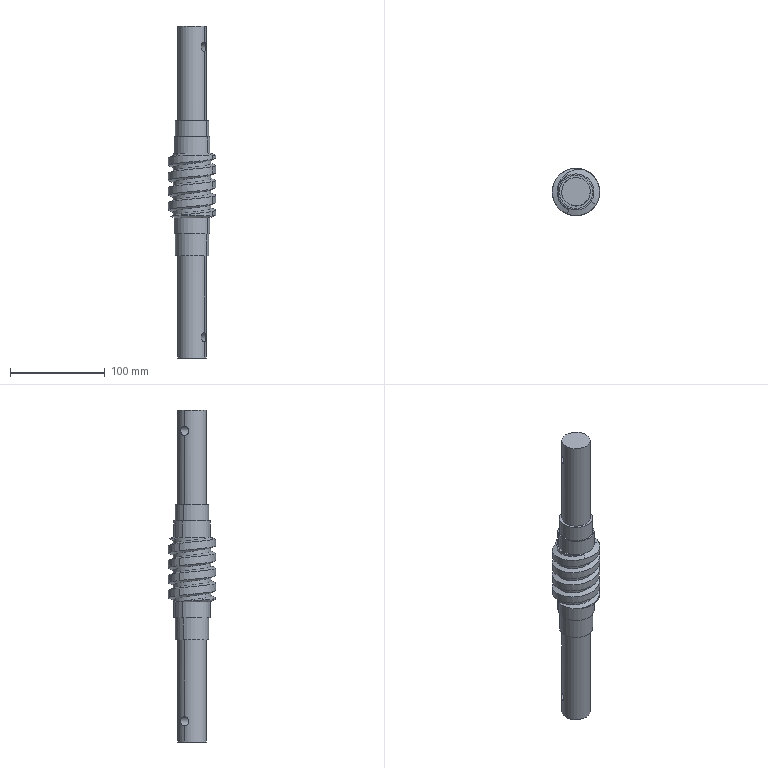Component | SolidWorks | 28-1 | 1 solid | 39 faces | volume 333145 mm3 | cylinder 26 | plane 6 | cone 4 | spline 3 | commonest cylinder face diameters 50 x10 10 x4 30 x4 35 x4 38 x4